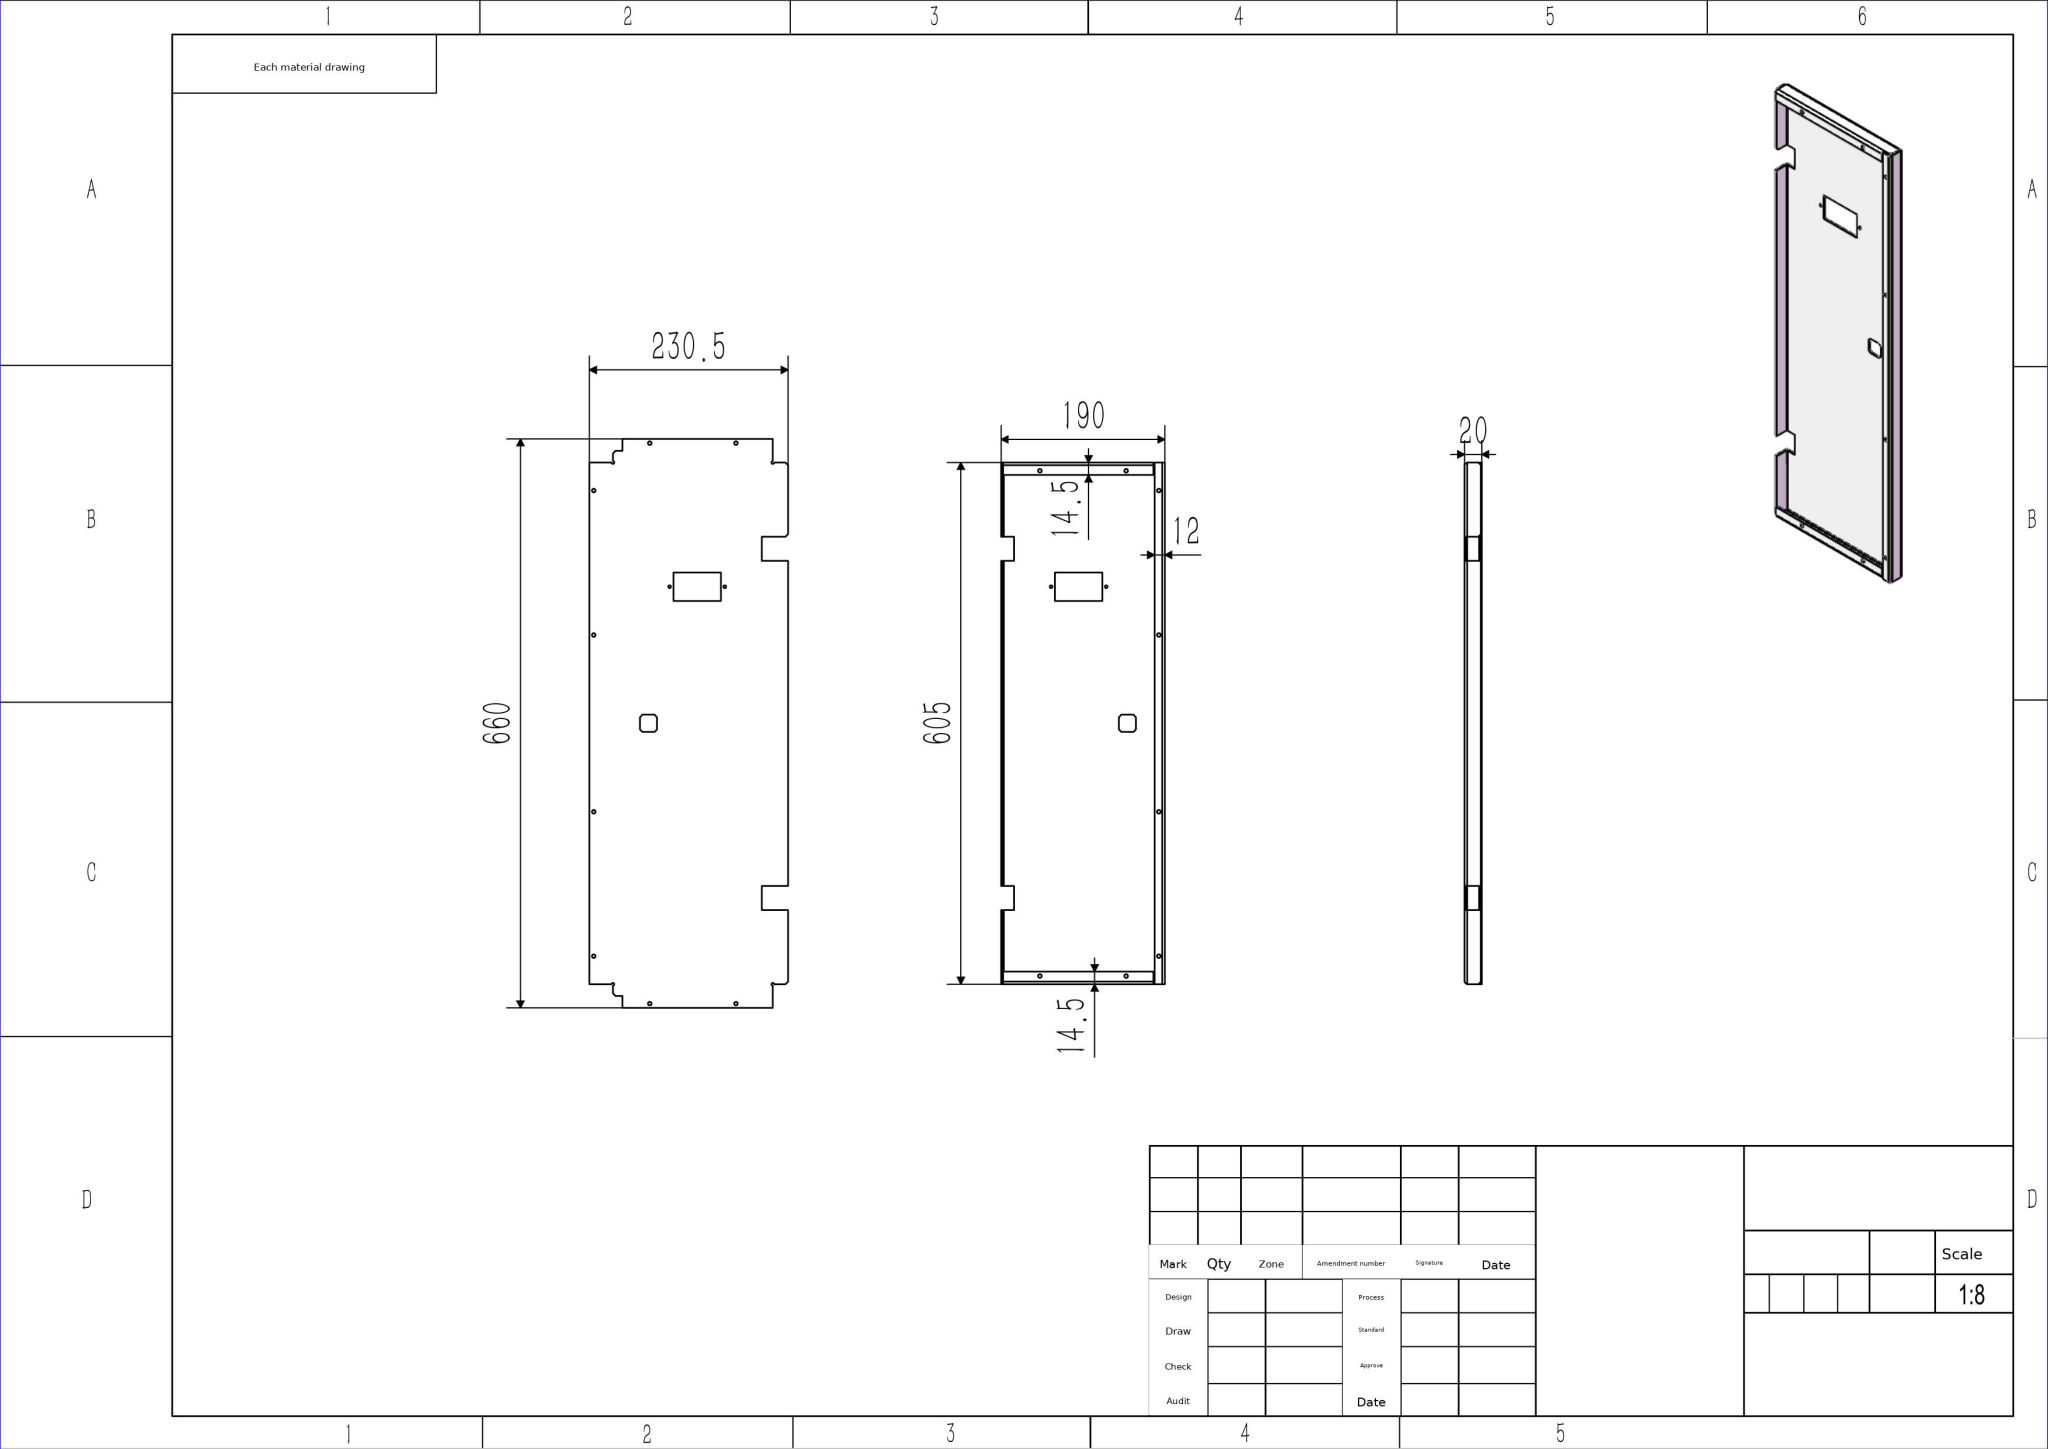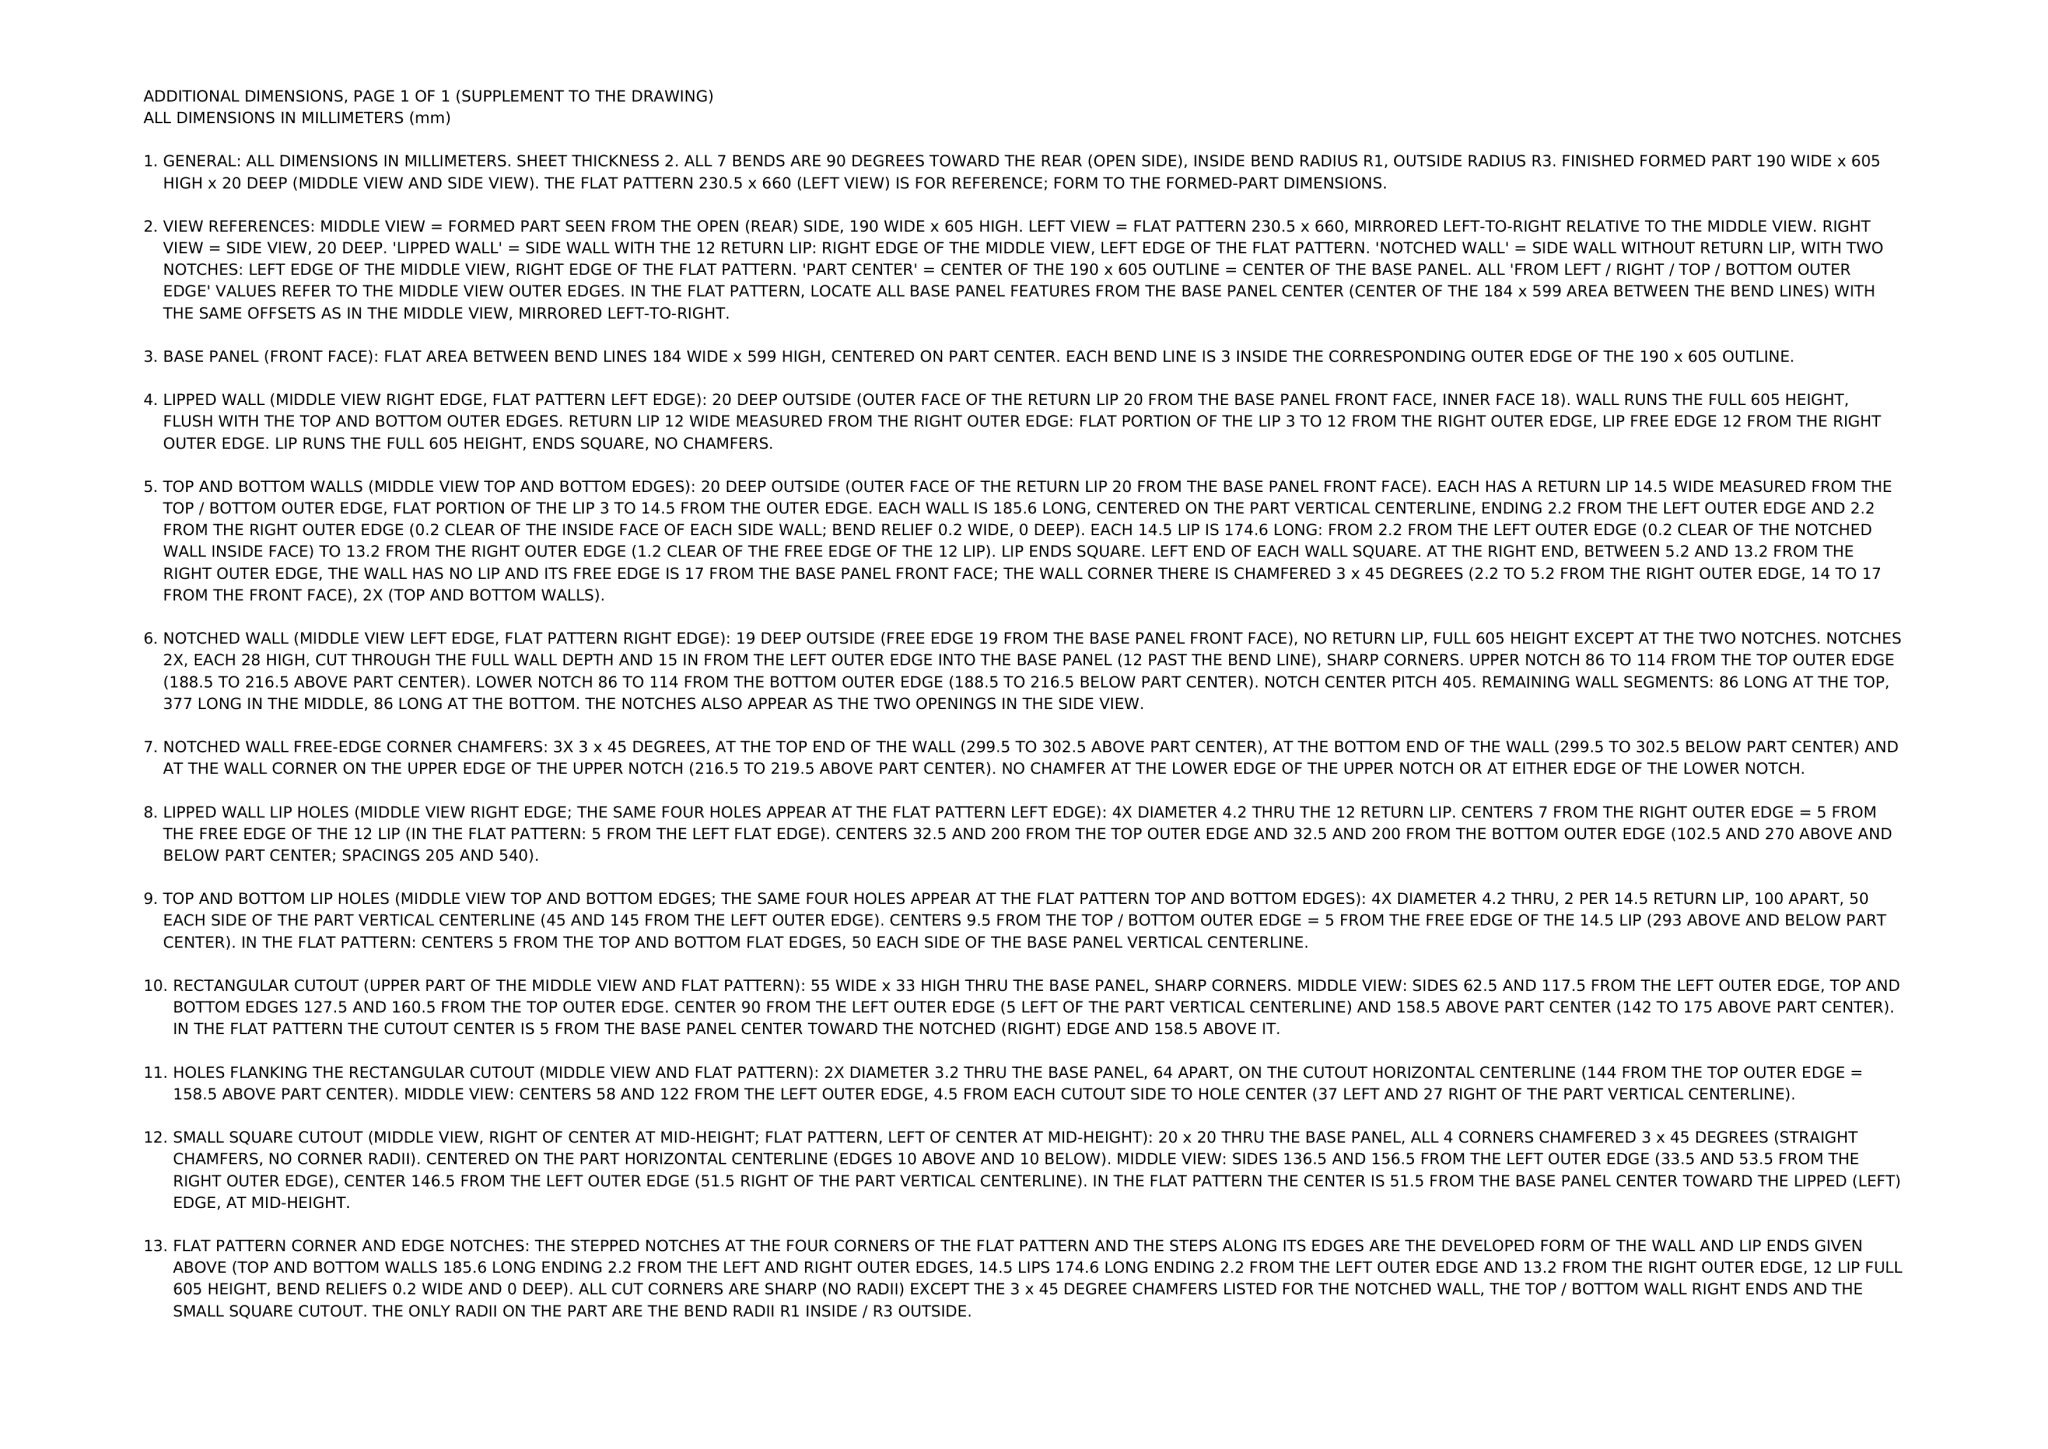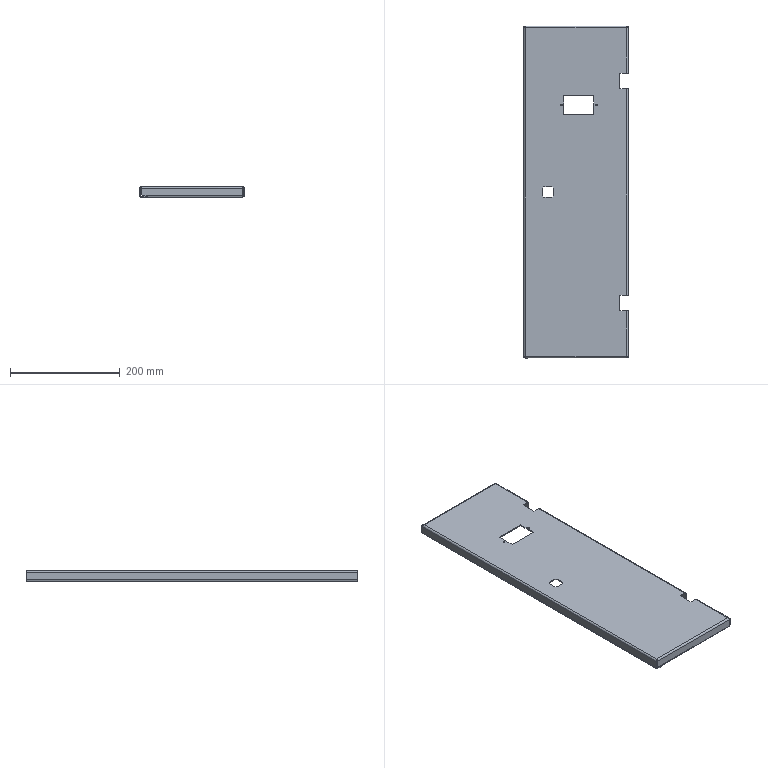Part | NX | mm | 1 solid | 117 faces | box 190 x 605 x 20 mm | volume 293749 mm3 | plane 71 | cylinder 38 | spline 8 | commonest cylinder face diameters 4.2 x16 2 x9 6 x9 3.2 x4